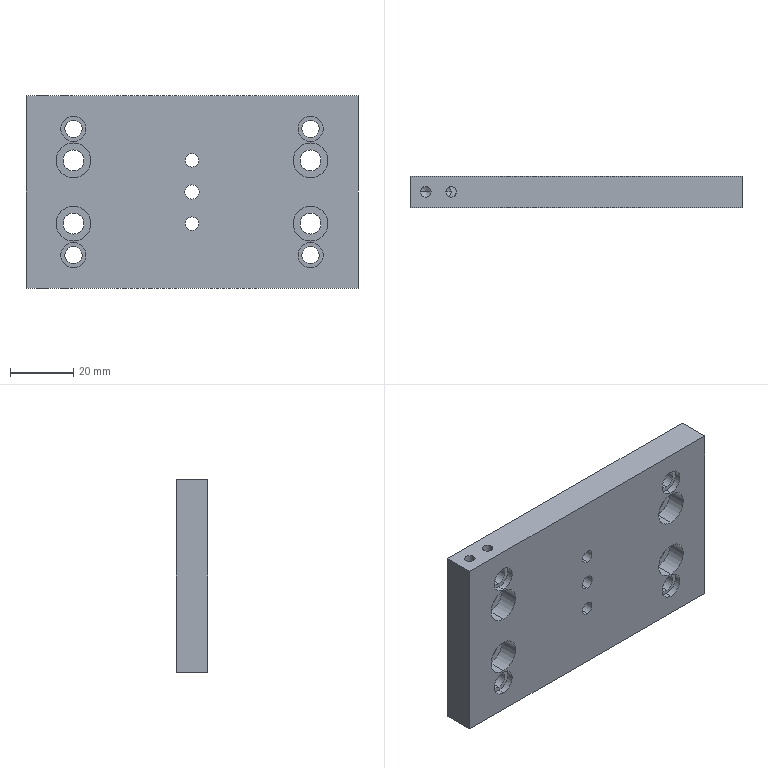Component | SolidWorks | F12529-M5102-1 | 1 solid | 83 faces | box 105 x 10 x 61 mm | volume 58770 mm3 | cylinder 56 | plane 19 | cone 8 | commonest cylinder face diameters 8 x10 3.3 x8 5.5 x8 11 x8 6.6 x8 10 x8 4.2 x4 4.5 x2
build123d program:
from build123d import *

# Parameters (mm, degrees)
SKETCH1_W                                            = 105
SKETCH1_H                                            = 61
EXTRUDE1_DEPTH                                       = 10
SKETCH3_R                                            = 4
CUT_EXTRUDE1_DEPTH                                   = 2
SKETCH5_R                                            = 5
CUT_EXTRUDE3_DEPTH                                   = 2
M6_HEX_SOCKET_HEAD_CAP_SCREW_COUNTERBORE_D           = 6.6
M6_HEX_SOCKET_HEAD_CAP_SCREW_COUNTERBORE_CBORE_D     = 11
M6_HEX_SOCKET_HEAD_CAP_SCREW_COUNTERBORE_CBORE_DEPTH = 6
SKETCH10_R                                           = 2.75
CUT_EXTRUDE4_DEPTH                                   = 10
M5_TAPPED_HOLE2_D                                    = 4.2
M5_TAPPED_HOLE2_DEPTH                                = 14
M5_TAPPED_HOLE2_TIP                                  = 1.262
COUNTERBORE_FOR_M4_HEX_SOCKET_HEAD_CAP_S_D           = 4.5
COUNTERBORE_FOR_M4_HEX_SOCKET_HEAD_CAP_S_CBORE_D     = 8
COUNTERBORE_FOR_M4_HEX_SOCKET_HEAD_CAP_S_CBORE_DEPTH = 4
M4_TAPPED_HOLE1_AT_2_COUNT                           = 2
M4_TAPPED_HOLE1_AT_2_PITCH                           = 8


with BuildPart() as part:
    # Sketch1 → Extrude1 (new body)
    with BuildSketch(Plane(origin=(0, 0, 0), x_dir=(1, 0, 0), z_dir=(0, 1, 0))):
        Rectangle(SKETCH1_W, SKETCH1_H)
    extrude(amount=EXTRUDE1_DEPTH)

    # Sketch3 → Cut-Extrude1 (cut)
    with BuildSketch(Plane(origin=(0, 0, 0), x_dir=(1, 0, 0), z_dir=(0, 1, 0))):
        with Locations(Location((37.5, 20, 0), (0, 0, 270))):
            Circle(SKETCH3_R)
        with Locations(Location((37.5, -20, 0), (0, 0, 270))):
            Circle(SKETCH3_R)
    cut_extrude1 = extrude(amount=CUT_EXTRUDE1_DEPTH, mode=Mode.SUBTRACT)

    # Mirror1: Cut-Extrude1 across plane
    add(cut_extrude1.mirror(Plane(origin=(0, 0, 0), x_dir=(0, 0, 1), z_dir=(1, 0, 0))), mode=Mode.SUBTRACT)

    # Sketch5 → Cut-Extrude3 (cut)
    with BuildSketch(Plane(origin=(0, 10, 0), x_dir=(1, 0, 0), z_dir=(0, 1, 0))):
        with Locations(Location((-37.5, -10, 0), (0, 0, 270))):
            Circle(SKETCH5_R)
        with Locations(Location((-37.5, 10, 0), (0, 0, 270))):
            Circle(SKETCH5_R)
    cut_extrude3 = extrude(amount=-CUT_EXTRUDE3_DEPTH, mode=Mode.SUBTRACT)

    # Mirror3: Cut-Extrude3 across plane
    add(cut_extrude3.mirror(Plane(origin=(0, 0, 0), x_dir=(0, 0, 1), z_dir=(1, 0, 0))), mode=Mode.SUBTRACT)

    # M6 Hex Socket Head Cap Screw Counterbore (through all)
    with Locations(Plane.XZ):
        with Locations((37.5, 10), (37.5, -10)):
            m6_hex_socket_head_cap_screw_counterbore = CounterBoreHole(M6_HEX_SOCKET_HEAD_CAP_SCREW_COUNTERBORE_D / 2, M6_HEX_SOCKET_HEAD_CAP_SCREW_COUNTERBORE_CBORE_D / 2, M6_HEX_SOCKET_HEAD_CAP_SCREW_COUNTERBORE_CBORE_DEPTH)

    # Mirror4: M6 Hex Socket Head Cap Screw Counterbore across plane
    add(m6_hex_socket_head_cap_screw_counterbore.mirror(Plane(origin=(0, 0, 0), x_dir=(0, 0, 1), z_dir=(1, 0, 0))), mode=Mode.SUBTRACT)

    # Sketch10 → Cut-Extrude4 (cut)
    with BuildSketch(Plane(origin=(0, 10, 0), x_dir=(1, 0, 0), z_dir=(0, 1, 0))):
        with Locations(Location((37.5, 20, 0), (0, 0, 270))):
            Circle(SKETCH10_R)
        with Locations(Location((37.5, -20, 0), (0, 0, 270))):
            Circle(SKETCH10_R)
    cut_extrude4 = extrude(amount=-CUT_EXTRUDE4_DEPTH, mode=Mode.SUBTRACT)

    # Mirror5: Cut-Extrude4 across plane
    add(cut_extrude4.mirror(Plane(origin=(0, 0, 0), x_dir=(0, 0, 1), z_dir=(1, 0, 0))), mode=Mode.SUBTRACT)

    # M5 Tapped Hole2
    with Locations(Plane(origin=(0, 10, 0), x_dir=(-1, 0, 0), z_dir=(0, 1, 0))):
        with Locations((0, -10), (0, 10)):
            Hole(M5_TAPPED_HOLE2_D / 2, depth=M5_TAPPED_HOLE2_DEPTH)
            with Locations((0, 0, -(M5_TAPPED_HOLE2_DEPTH + M5_TAPPED_HOLE2_TIP / 2))):  # 118° drill point
                Cone(0, M5_TAPPED_HOLE2_D / 2, M5_TAPPED_HOLE2_TIP, mode=Mode.SUBTRACT)

    # Counterbore for M4 Hex Socket Head Cap S (through all)
    with Locations(Plane(origin=(0, 10, 0), x_dir=(-1, 0, 0), z_dir=(0, 1, 0))):
        with Locations((0, 0)):
            CounterBoreHole(COUNTERBORE_FOR_M4_HEX_SOCKET_HEAD_CAP_S_D / 2, COUNTERBORE_FOR_M4_HEX_SOCKET_HEAD_CAP_S_CBORE_D / 2, COUNTERBORE_FOR_M4_HEX_SOCKET_HEAD_CAP_S_CBORE_DEPTH)

    # Sketch15 → M4 Tapped Hole1 (revolve, cut)
    with BuildSketch(Plane(origin=(-39.5, 5, 30.5), x_dir=(0, -1, 0), z_dir=(1, 0, 0))):
        Polygon((0, 0), (0, 12.491), (1.65, 11.5), (1.65, 0), align=None)
    m4_tapped_hole1 = revolve(axis=Axis((-39.5, 5, 36.85), (0, 0, -1)), mode=Mode.SUBTRACT)

    # M4 Tapped Hole1 at 2: M4 Tapped Hole1 ×2
    with Locations(*[(-i * M4_TAPPED_HOLE1_AT_2_PITCH, 0, 0) for i in range(1, M4_TAPPED_HOLE1_AT_2_COUNT)]):
        add(m4_tapped_hole1, mode=Mode.SUBTRACT)

    # Mirror6: M4 Tapped Hole1 across plane
    add(m4_tapped_hole1.mirror(Plane.XY), mode=Mode.SUBTRACT)

    # Mirror6 copy 1 sketch → Mirror6 copy 1 (revolve, cut)
    with BuildSketch(Plane(origin=(-47.5, 5, -30.5), x_dir=(0, -1, 0), z_dir=(1, 0, 0))):
        Polygon((0, 0), (0, -12.491), (1.65, -11.5), (1.65, 0), align=None)
    revolve(axis=Axis((-47.5, 5, -36.85), (0, 0, -1)), mode=Mode.SUBTRACT)


solid = part.part

# Placed as in the assembly
solid = solid.moved(Location((0, 193, 0), (0, 0, 0)))